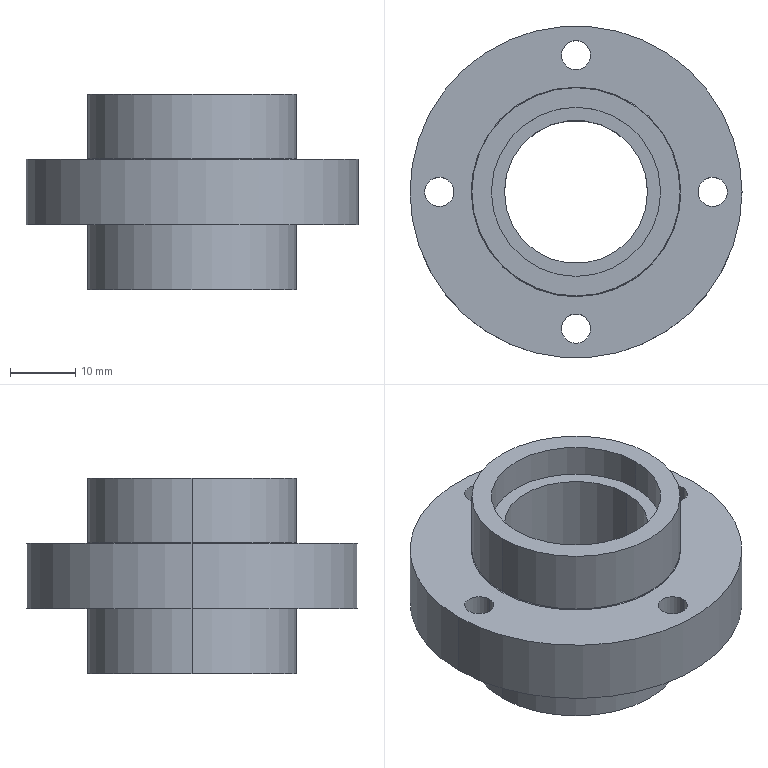Component | SolidWorks | 170423A4-ConveyorSynchronousPulleyAssembly-1_170423A4-BFY01-6803ZZ-L30-1_170423A4-HI_BFY01-6803ZZ-L30S-1 | 1 solid | 40 faces | volume 22402 mm3 | cylinder 28 | plane 10 | spline 2 | commonest cylinder face diameters 8 x8 4.5 x8 32 x4 26 x4 51 x2 22 x2